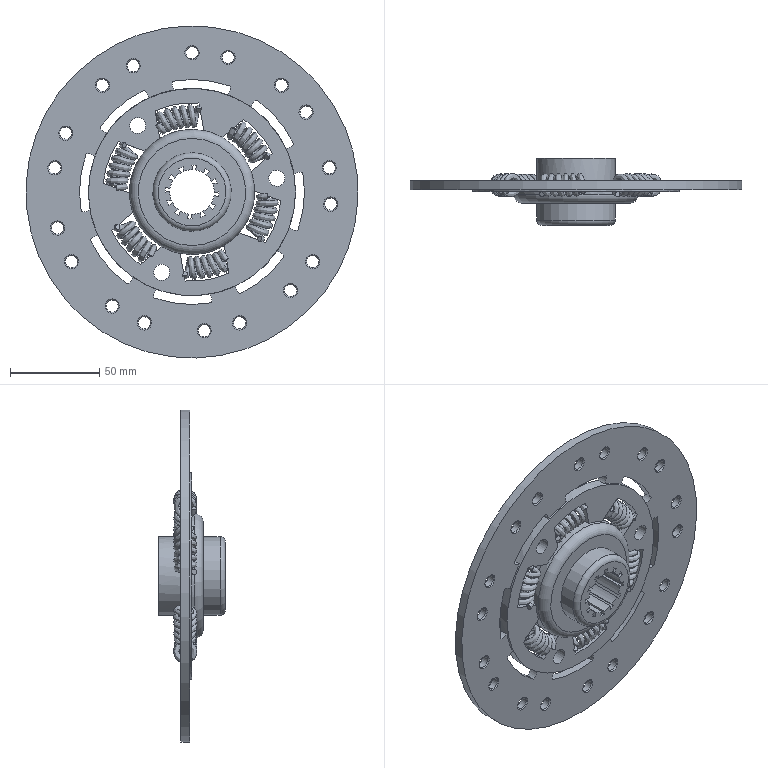Component | NX | SPRING_PRESSURE_FRICTION_PLATE | 1 solid | 196 faces | volume 170303 mm3 | cylinder 86 | plane 66 | cone 36 | spline 6 | torus 2 | commonest cylinder face diameters 6.8 x18 10.114 x16 30 x12 25 x12 126 x8 70 x6 100 x6 9 x3